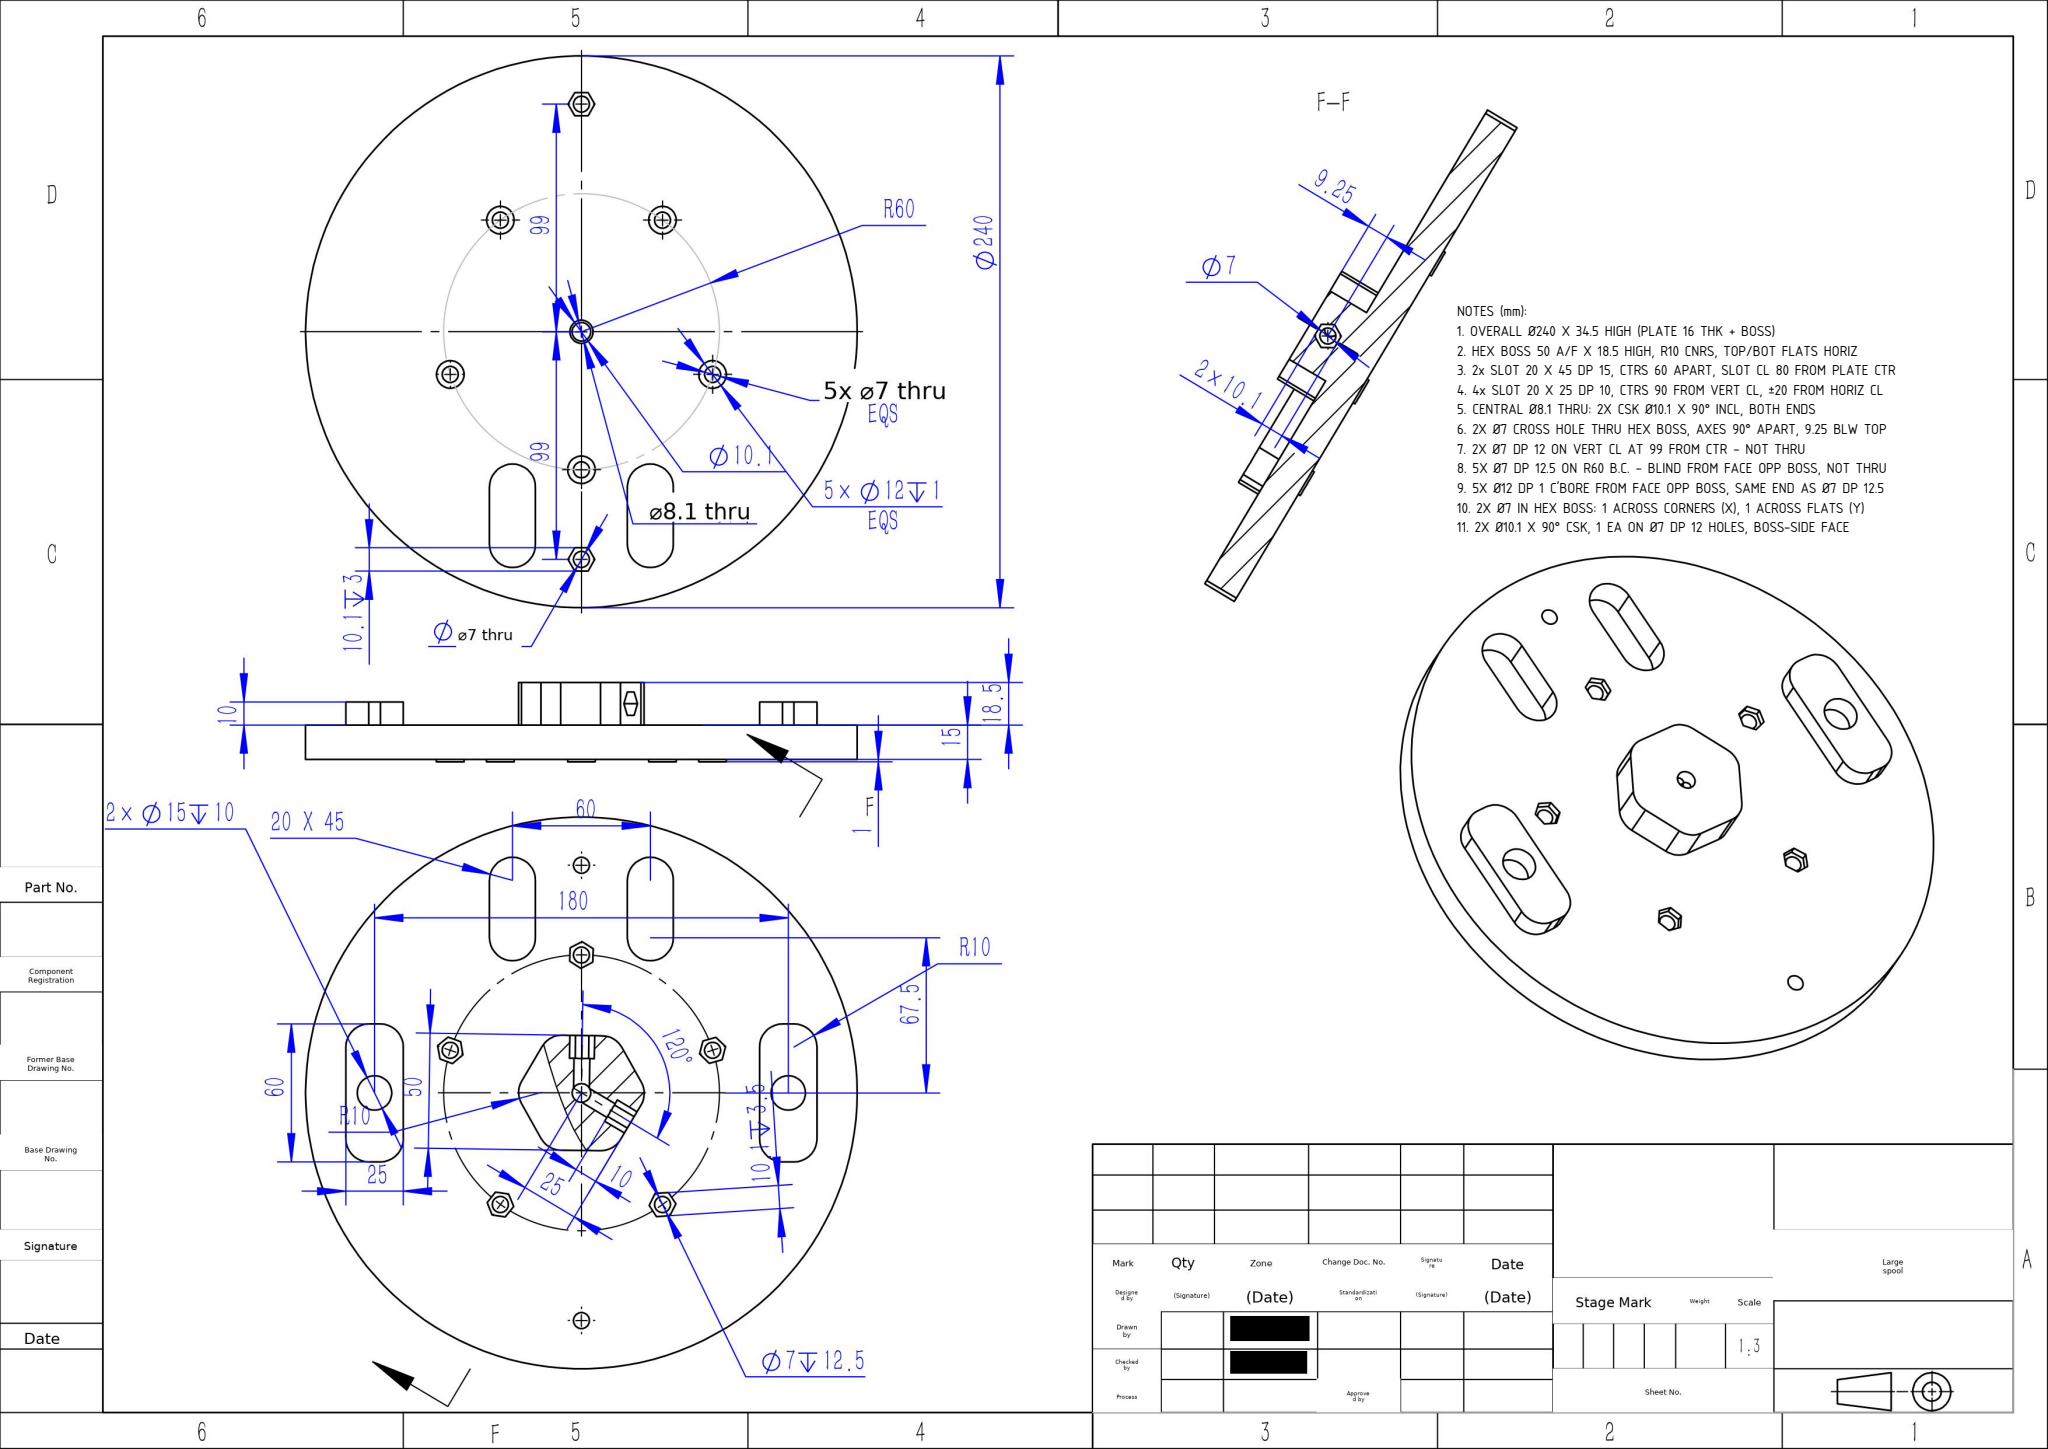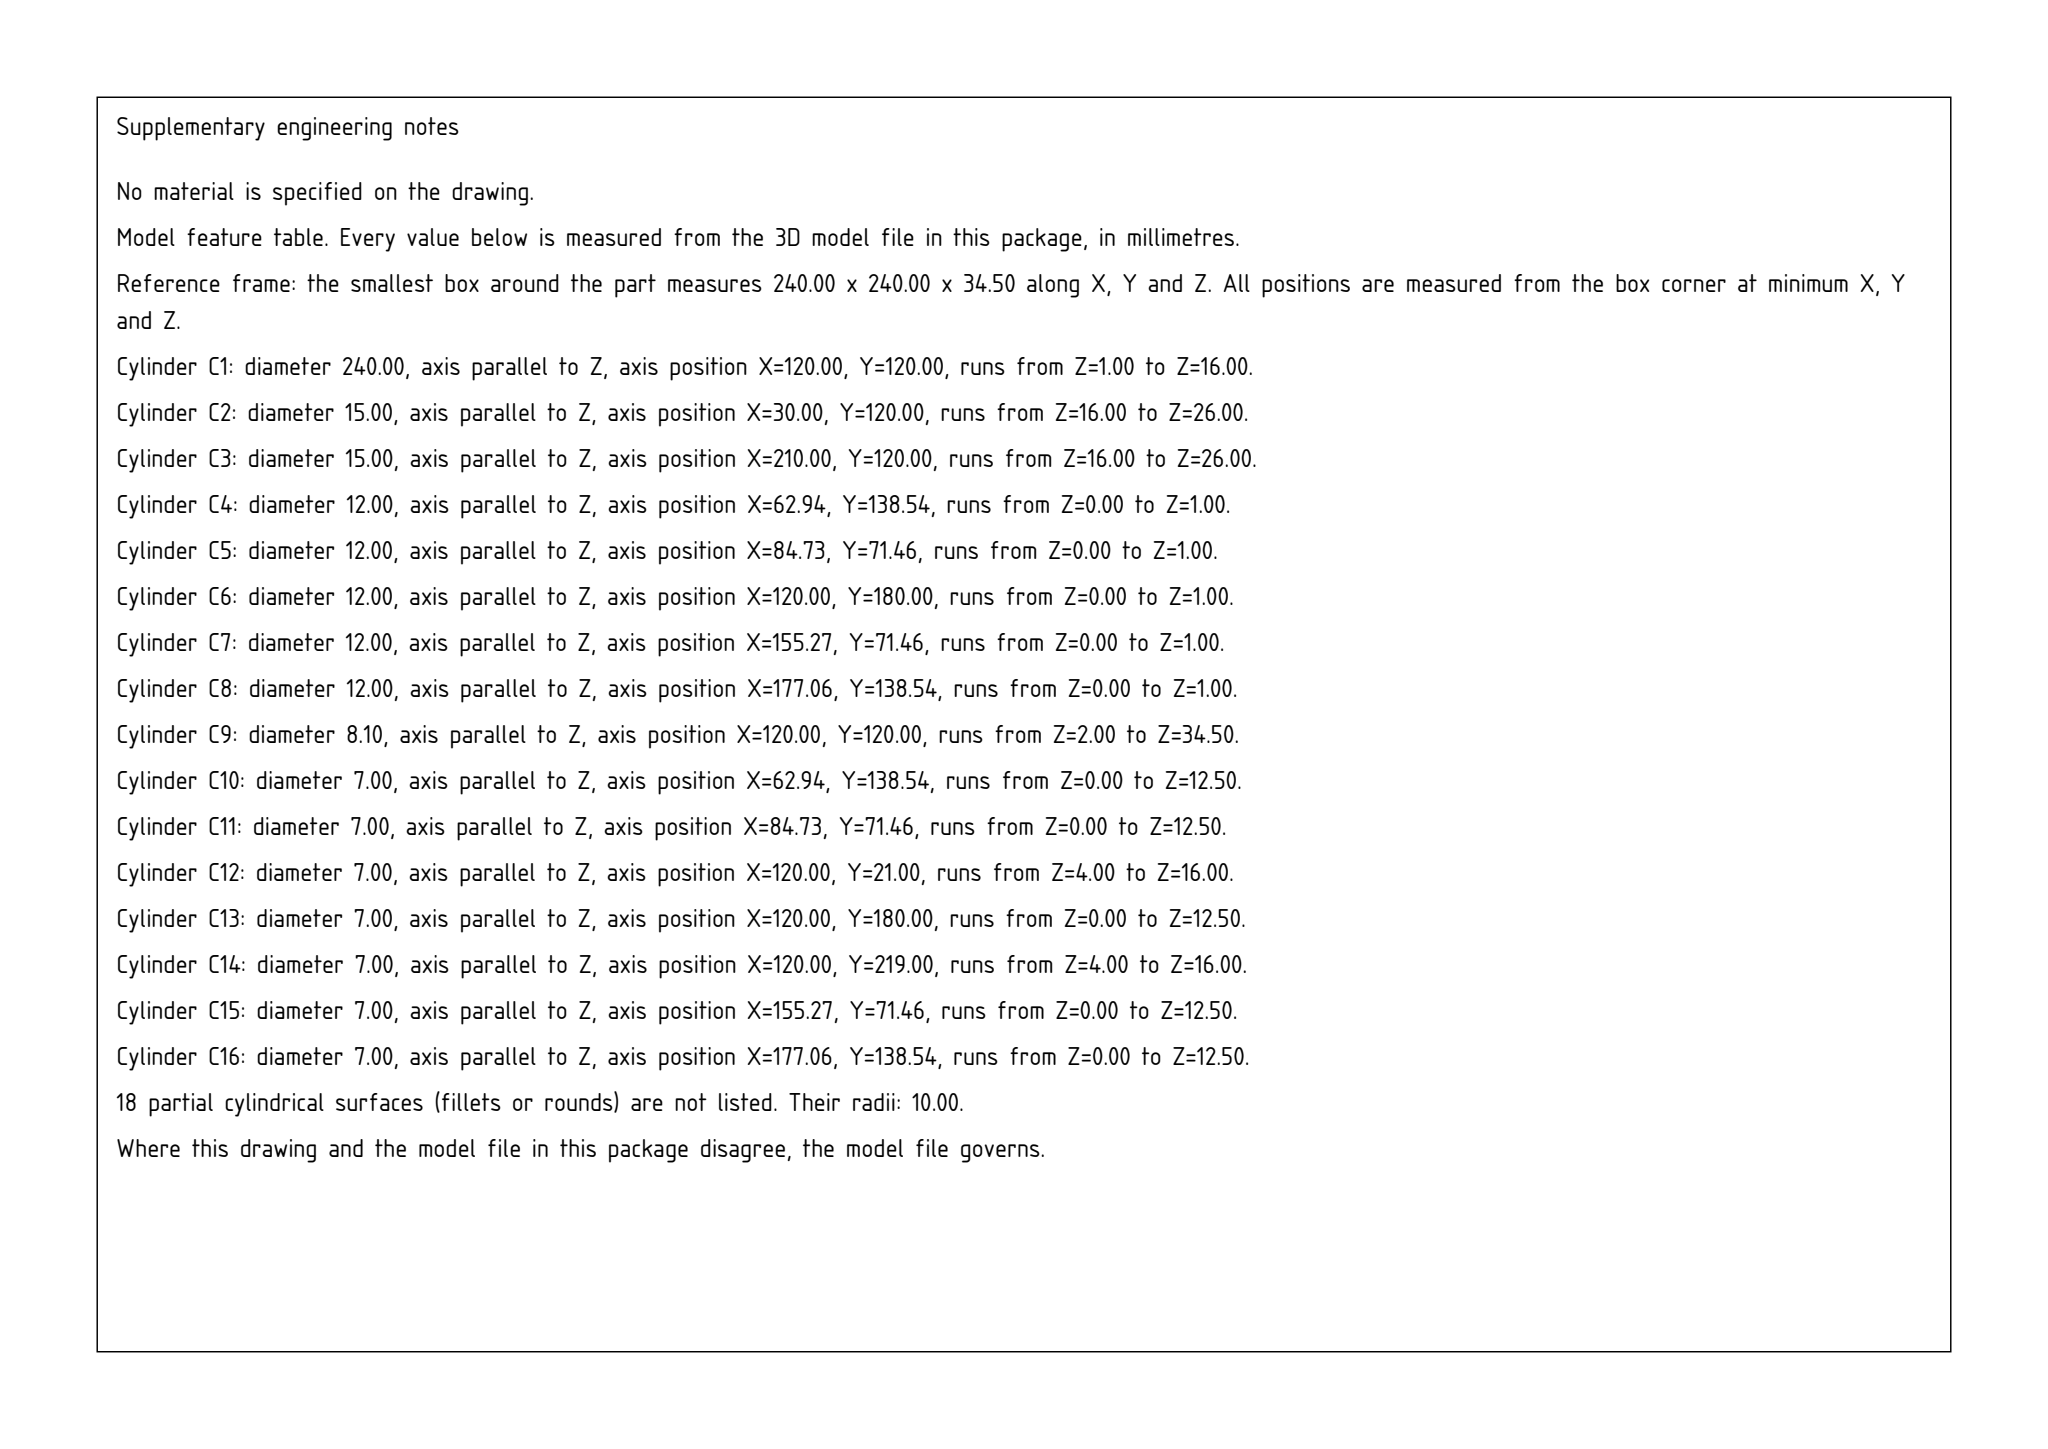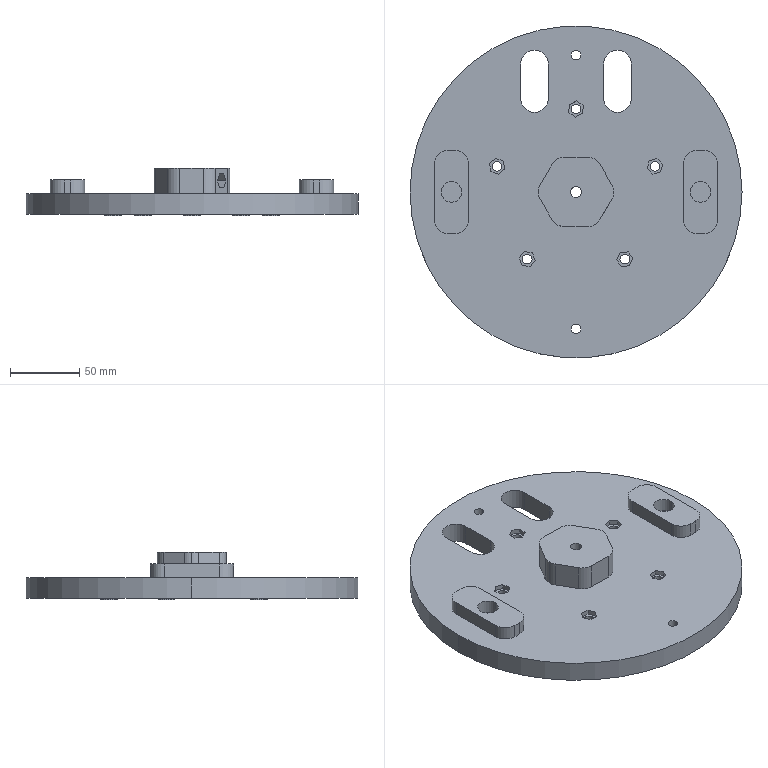Part | SolidWorks | mm | 1 solid | 150 faces | box 240 x 240 x 34.5 mm | volume 709143 mm3 | plane 93 | cylinder 55 | cone 2 | commonest cylinder face diameters 20 x19 7 x18 12 x10 15 x4 8.1 x2 240 x2
Drawing notes:
OVERALL Ø240 X 34.5 HIGH (PLATE 16 THK + BOSS) | from the solid: bbox 240x240x34.5; z planes 0/16/34.5, dia240 cyl len 15/16 base
HEX BOSS 50 A/F X 18.5 HIGH, R10 CNRS, TOP/BOT FLATS HORIZ | from the solid: 6x R10 cnr cyls Ø20 len18.5 at r=17.32 from (120,120), 0/60/120°; 2*(17.32*cos30+10)=50 A/F; boss top z=34.5
2x SLOT 20 X 45 DP 15, CTRS 60 APART, SLOT CL 80 FROM PLATE CTR | from the solid: Ø20 len15 ends (90,187.5)(90,212.5)(150,187.5)(150,212.5): 20 wide x 45 long, ctr y=200, x 90/150
4x SLOT 20 X 25 DP 10, CTRS 90 FROM VERT CL, ±20 FROM HORIZ CL | from the solid: Ø20 len10 ends x=27.5/32.5 & 207.5/212.5 at y=100 & 140: ctrs (30,100)(30,140)(210,100)(210,140)
CENTRAL Ø8.1 THRU: 2X CSK Ø10.1 X 90° INCL, BOTH ENDS | from the solid: cones[included_angle,ref_dia]=[[90.0,10.1,2]] on Ø8.1 z-hole at (120,120), len 32.5
2X Ø7 CROSS HOLE THRU HEX BOSS, AXES 90° APART, 9.25 BLW TOP | from the solid: Ø7 axis x at z=25.25 (2 faces) + Ø7 axis y at x=118.21, z=25.25 (2 faces); top face z=34.5, 34.5-25.25=9.25
2X Ø7 DP 12 ON VERT CL AT 99 FROM CTR - NOT THRU | from the solid: Ø7 axis z at (120,21) and (120,219), length 12.0; centre (120,120) => 99 offset
5X Ø7 DP 12.5 ON R60 B.C. - BLIND FROM FACE OPP BOSS, NOT THRU | from the solid: Ø7 z-axis cyls at R60 (62.94/84.73/120,180/155.27/177.06) length 12.5, z 0-12.5 in 16 thk plate
5X Ø12 DP 1 C'BORE FROM FACE OPP BOSS, SAME END AS Ø7 DP 12.5 | from the solid: Ø12 z-cyls len 1.0 at same R60 positions, z-plane at 1.0 (face z=0); boss runs z=16-34.5
2X Ø7 IN HEX BOSS: 1 ACROSS CORNERS (X), 1 ACROSS FLATS (Y) | from the solid: Ø7 axis-x and axis-y holes at z=25.25 (9.25 above z=16 boss base); hex corner cyls at 102.68/137.32 on X
2X Ø10.1 X 90° CSK, 1 EA ON Ø7 DP 12 HOLES, BOSS-SIDE FACE | from the solid: cones[90°, ref dia 10.1] count 2; Ø7 z-holes at (120,21) & (120,219) len 12, z 4-16